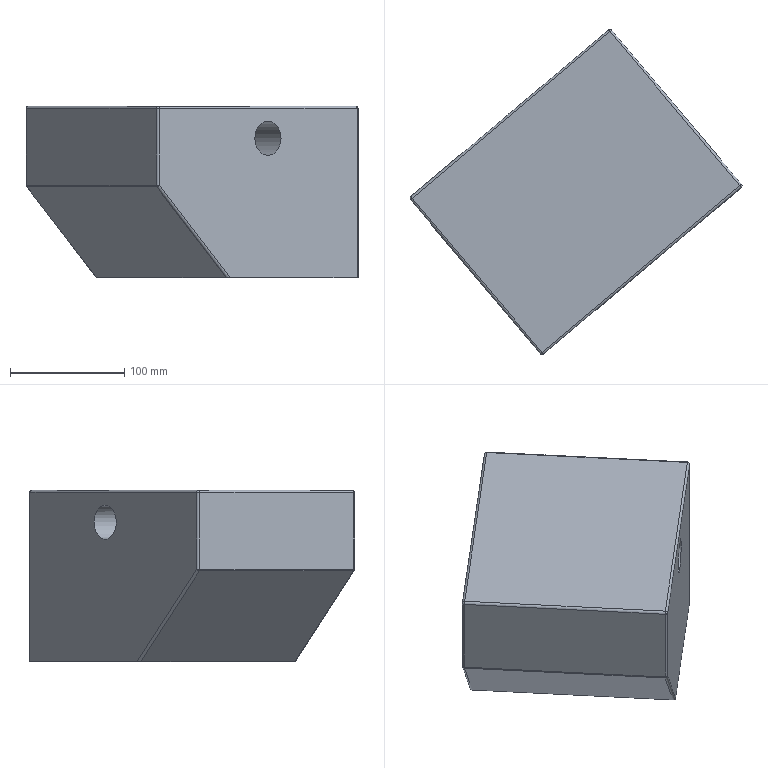Component | NX | BASEUP | 1 solid | 27 faces | volume 5316905 mm3 | cylinder 13 | plane 8 | sphere 6 | commonest cylinder face diameters 4 x11 98 x1 30 x1